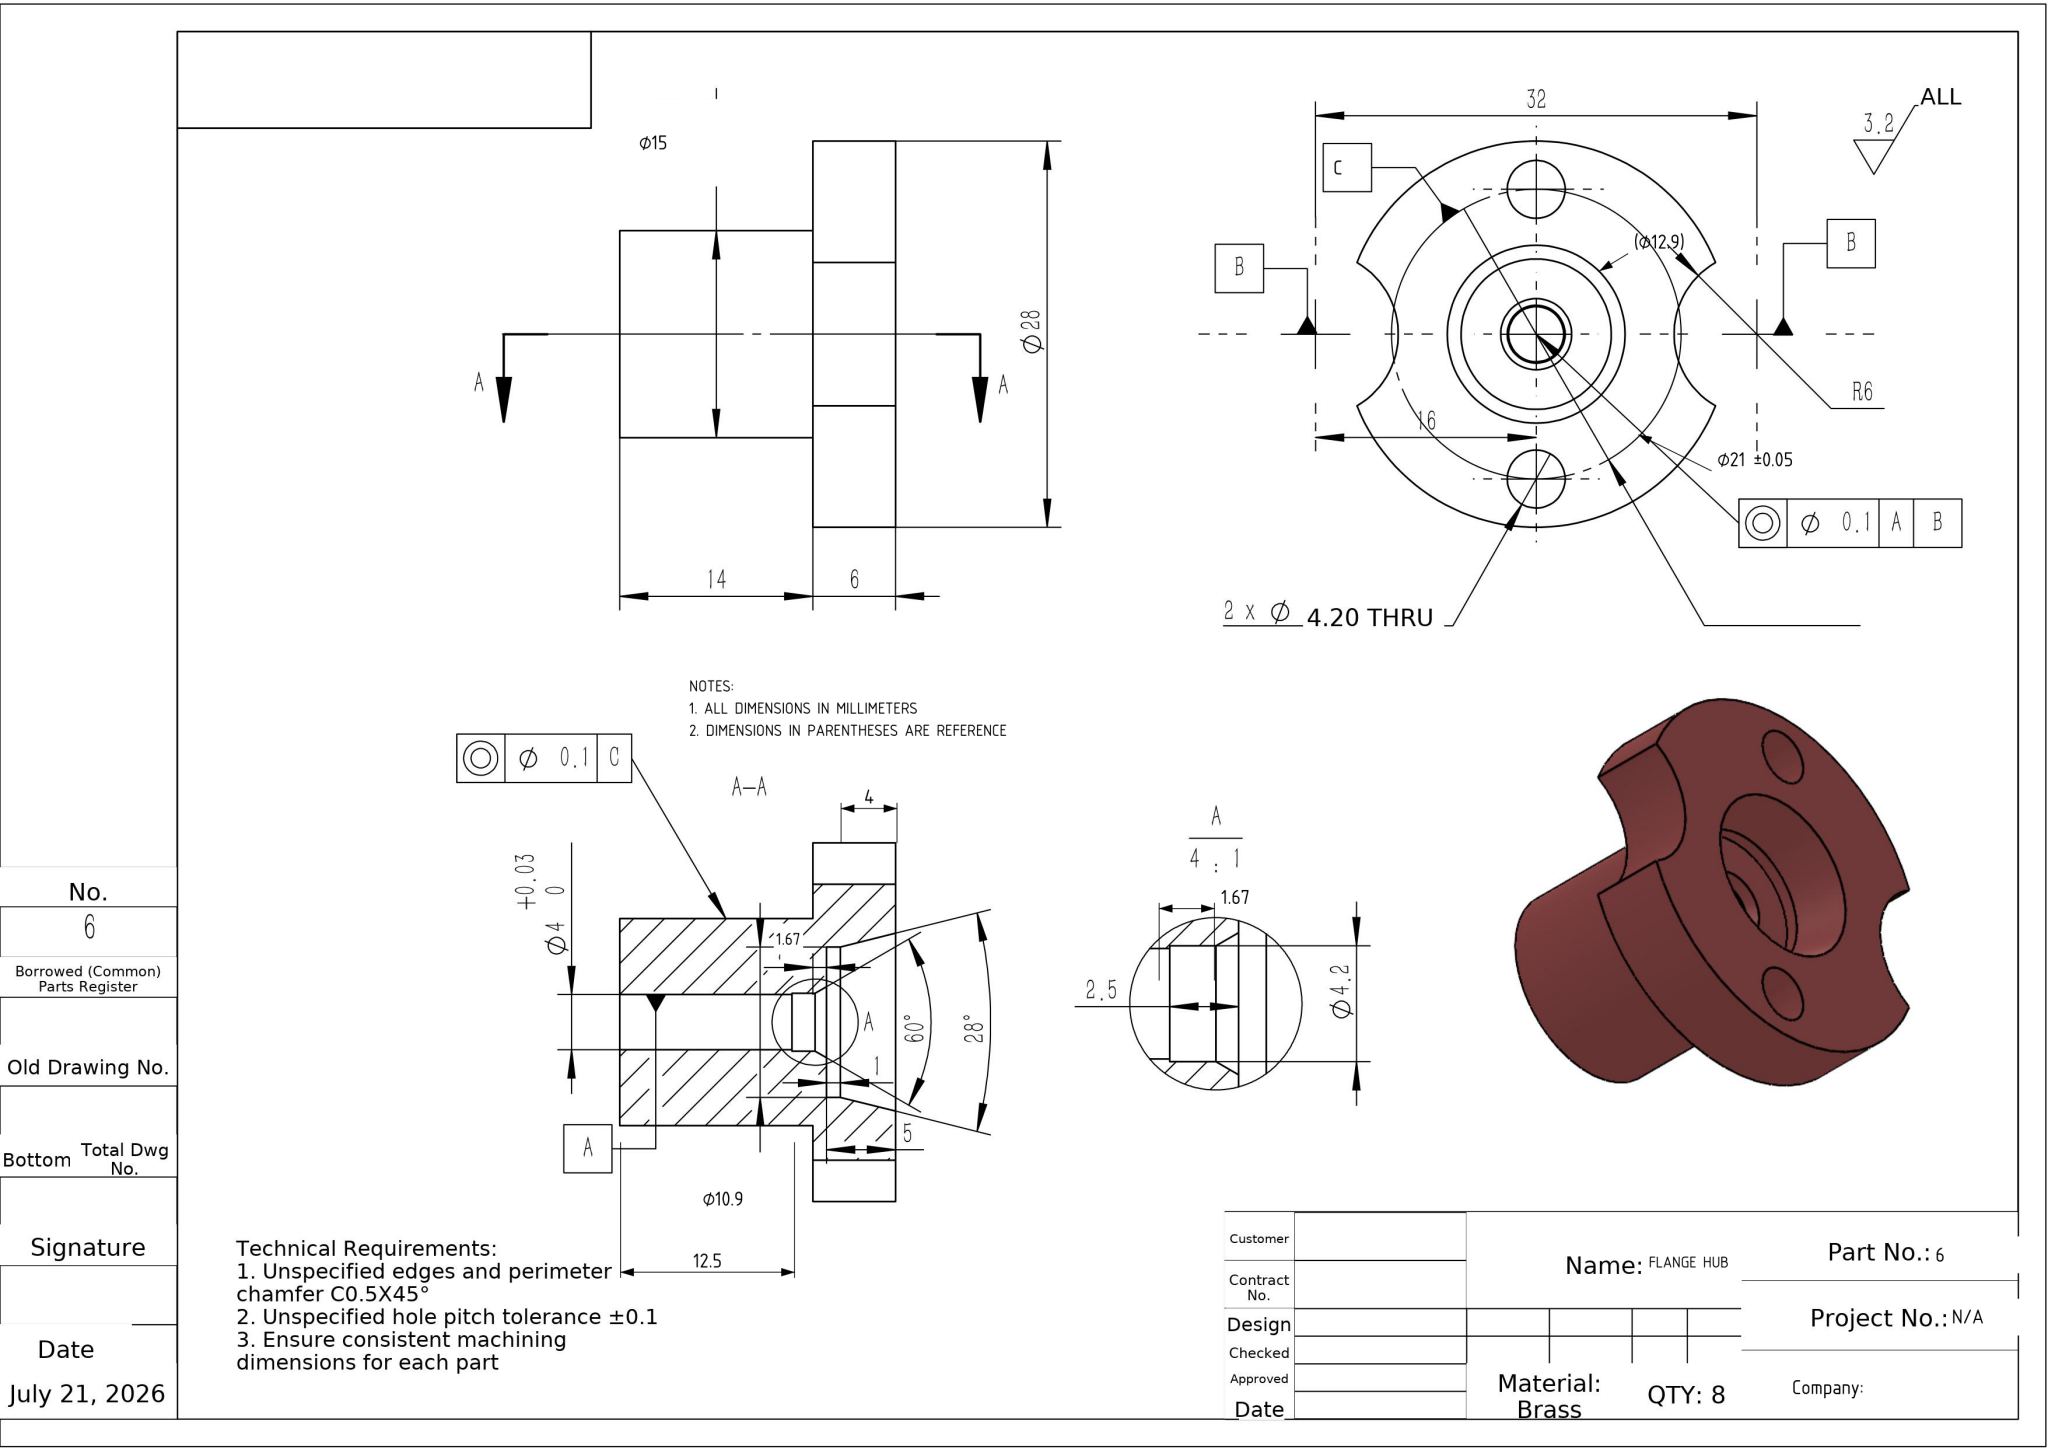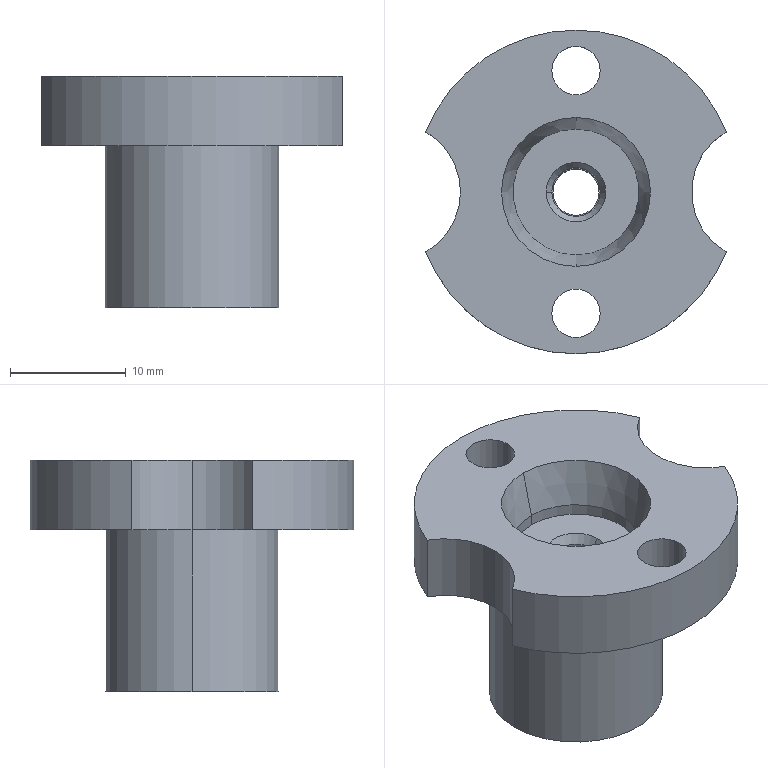Part | NX | mm | 1 solid | 26 faces | box 26 x 28 x 20 mm | volume 4920 mm3 | cylinder 17 | plane 5 | cone 4 | commonest cylinder face diameters 4.2 x6 12 x3 10.9 x2 15 x2 4 x2 28 x2
STEP:
#1=CARTESIAN_POINT('',(-2.1,0.,14.5));
#2=VERTEX_POINT('',#1);
#3=CARTESIAN_POINT('',(2.1,0.,14.5));
#4=VERTEX_POINT('',#3);
#5=CARTESIAN_POINT('',(0.,0.,14.5));
#6=DIRECTION('',(0.,0.,1.));
#7=DIRECTION('',(1.,0.,0.));
#8=AXIS2_PLACEMENT_3D('',#5,#6,#7);
#9=CIRCLE('',#8,2.1);
#10=EDGE_CURVE('',#2,#4,#9,.T.);
#11=ORIENTED_EDGE('',*,*,#10,.F.);
#12=CARTESIAN_POINT('',(-2.1,0.,16.173));
#13=VERTEX_POINT('',#12);
#14=CARTESIAN_POINT('',(-2.1,0.,14.5));
#15=DIRECTION('',(0.,0.,1.));
#16=VECTOR('',#15,1000.);
#17=LINE('',#14,#16);
#18=EDGE_CURVE('',#2,#13,#17,.T.);
#19=ORIENTED_EDGE('',*,*,#18,.T.);
#20=CARTESIAN_POINT('',(2.1,0.,16.173));
#21=VERTEX_POINT('',#20);
#22=CARTESIAN_POINT('',(0.,0.,16.173));
#23=DIRECTION('',(0.,0.,-1.));
#24=DIRECTION('',(1.,0.,0.));
#25=AXIS2_PLACEMENT_3D('',#22,#23,#24);
#26=CIRCLE('',#25,2.1);
#27=EDGE_CURVE('',#21,#13,#26,.T.);
#28=ORIENTED_EDGE('',*,*,#27,.F.);
#29=CARTESIAN_POINT('',(2.1,0.,14.5));
#30=DIRECTION('',(0.,0.,1.));
#31=VECTOR('',#30,1000.);
#32=LINE('',#29,#31);
#33=EDGE_CURVE('',#4,#21,#32,.T.);
#34=ORIENTED_EDGE('',*,*,#33,.F.);
#35=EDGE_LOOP('',(#11,#19,#28,#34));
#36=FACE_OUTER_BOUND('',#35,.T.);
#37=CARTESIAN_POINT('',(0.,0.,14.5));
#38=DIRECTION('',(0.,0.,1.));
#39=DIRECTION('',(1.,0.,0.));
#40=AXIS2_PLACEMENT_3D('',#37,#38,#39);
#41=CYLINDRICAL_SURFACE('',#40,2.1);
#42=ADVANCED_FACE('',(#36),#41,.F.);
#43=CARTESIAN_POINT('',(-13.,5.196,16.));
#44=VERTEX_POINT('',#43);
#45=CARTESIAN_POINT('',(-10.,0.,16.));
#46=VERTEX_POINT('',#45);
#47=CARTESIAN_POINT('',(-16.,0.,16.));
#48=DIRECTION('',(0.,0.,-1.));
#49=DIRECTION('',(-1.,0.,0.));
#50=AXIS2_PLACEMENT_3D('',#47,#48,#49);
#51=CIRCLE('',#50,6.);
#52=EDGE_CURVE('',#44,#46,#51,.T.);
#53=ORIENTED_EDGE('',*,*,#52,.T.);
#54=CARTESIAN_POINT('',(-10.,0.,22.));
#55=VERTEX_POINT('',#54);
#56=CARTESIAN_POINT('',(-10.,0.,0.));
#57=DIRECTION('',(0.,0.,1.));
#58=VECTOR('',#57,1000.);
#59=LINE('',#56,#58);
#60=EDGE_CURVE('',#46,#55,#59,.T.);
#61=ORIENTED_EDGE('',*,*,#60,.T.);
#62=CARTESIAN_POINT('',(-13.,5.196,22.));
#63=VERTEX_POINT('',#62);
#64=CARTESIAN_POINT('',(-16.,0.,22.));
#65=DIRECTION('',(0.,0.,1.));
#66=DIRECTION('',(1.,0.,0.));
#67=AXIS2_PLACEMENT_3D('',#64,#65,#66);
#68=CIRCLE('',#67,6.);
#69=EDGE_CURVE('',#55,#63,#68,.T.);
#70=ORIENTED_EDGE('',*,*,#69,.T.);
#71=CARTESIAN_POINT('',(-13.,5.196,11.));
#72=DIRECTION('',(0.,0.,1.));
#73=VECTOR('',#72,1000.);
#74=LINE('',#71,#73);
#75=EDGE_CURVE('',#44,#63,#74,.T.);
#76=ORIENTED_EDGE('',*,*,#75,.F.);
#77=EDGE_LOOP('',(#53,#61,#70,#76));
#78=FACE_OUTER_BOUND('',#77,.T.);
#79=CARTESIAN_POINT('',(-16.,0.,0.));
#80=DIRECTION('',(0.,0.,1.));
#81=DIRECTION('',(1.,0.,0.));
#82=AXIS2_PLACEMENT_3D('',#79,#80,#81);
#83=CYLINDRICAL_SURFACE('',#82,6.);
#84=ADVANCED_FACE('',(#78),#83,.F.);
#85=CARTESIAN_POINT('',(2.1,10.5,16.));
#86=VERTEX_POINT('',#85);
#87=CARTESIAN_POINT('',(-2.1,10.5,16.));
#88=VERTEX_POINT('',#87);
#89=CARTESIAN_POINT('',(0.,10.5,16.));
#90=DIRECTION('',(0.,0.,-1.));
#91=DIRECTION('',(-1.,0.,0.));
#92=AXIS2_PLACEMENT_3D('',#89,#90,#91);
#93=CIRCLE('',#92,2.1);
#94=EDGE_CURVE('',#86,#88,#93,.T.);
#95=ORIENTED_EDGE('',*,*,#94,.T.);
#96=CARTESIAN_POINT('',(-2.1,10.5,22.));
#97=VERTEX_POINT('',#96);
#98=CARTESIAN_POINT('',(-2.1,10.5,22.));
#99=DIRECTION('',(0.,0.,1.));
#100=VECTOR('',#99,1000.);
#101=LINE('',#98,#100);
#102=EDGE_CURVE('',#88,#97,#101,.T.);
#103=ORIENTED_EDGE('',*,*,#102,.T.);
#104=CARTESIAN_POINT('',(2.1,10.5,22.));
#105=VERTEX_POINT('',#104);
#106=CARTESIAN_POINT('',(0.,10.5,22.));
#107=DIRECTION('',(0.,0.,1.));
#108=DIRECTION('',(1.,0.,0.));
#109=AXIS2_PLACEMENT_3D('',#106,#107,#108);
#110=CIRCLE('',#109,2.1);
#111=EDGE_CURVE('',#97,#105,#110,.T.);
#112=ORIENTED_EDGE('',*,*,#111,.T.);
#113=CARTESIAN_POINT('',(2.1,10.5,22.));
#114=DIRECTION('',(0.,0.,1.));
#115=VECTOR('',#114,1000.);
#116=LINE('',#113,#115);
#117=EDGE_CURVE('',#86,#105,#116,.T.);
#118=ORIENTED_EDGE('',*,*,#117,.F.);
#119=EDGE_LOOP('',(#95,#103,#112,#118));
#120=FACE_OUTER_BOUND('',#119,.T.);
#121=CARTESIAN_POINT('',(0.,10.5,22.));
#122=DIRECTION('',(0.,0.,1.));
#123=DIRECTION('',(1.,0.,0.));
#124=AXIS2_PLACEMENT_3D('',#121,#122,#123);
#125=CYLINDRICAL_SURFACE('',#124,2.1);
#126=ADVANCED_FACE('',(#120),#125,.F.);
#127=CARTESIAN_POINT('',(2.1,-10.5,16.));
#128=VERTEX_POINT('',#127);
#129=CARTESIAN_POINT('',(-2.1,-10.5,16.));
#130=VERTEX_POINT('',#129);
#131=CARTESIAN_POINT('',(0.,-10.5,16.));
#132=DIRECTION('',(0.,0.,-1.));
#133=DIRECTION('',(-1.,0.,0.));
#134=AXIS2_PLACEMENT_3D('',#131,#132,#133);
#135=CIRCLE('',#134,2.1);
#136=EDGE_CURVE('',#128,#130,#135,.T.);
#137=ORIENTED_EDGE('',*,*,#136,.T.);
#138=CARTESIAN_POINT('',(-2.1,-10.5,22.));
#139=VERTEX_POINT('',#138);
#140=CARTESIAN_POINT('',(-2.1,-10.5,22.));
#141=DIRECTION('',(0.,0.,1.));
#142=VECTOR('',#141,1000.);
#143=LINE('',#140,#142);
#144=EDGE_CURVE('',#130,#139,#143,.T.);
#145=ORIENTED_EDGE('',*,*,#144,.T.);
#146=CARTESIAN_POINT('',(2.1,-10.5,22.));
#147=VERTEX_POINT('',#146);
#148=CARTESIAN_POINT('',(0.,-10.5,22.));
#149=DIRECTION('',(0.,0.,1.));
#150=DIRECTION('',(1.,0.,0.));
#151=AXIS2_PLACEMENT_3D('',#148,#149,#150);
#152=CIRCLE('',#151,2.1);
#153=EDGE_CURVE('',#139,#147,#152,.T.);
#154=ORIENTED_EDGE('',*,*,#153,.T.);
#155=CARTESIAN_POINT('',(2.1,-10.5,22.));
#156=DIRECTION('',(0.,0.,1.));
#157=VECTOR('',#156,1000.);
#158=LINE('',#155,#157);
#159=EDGE_CURVE('',#128,#147,#158,.T.);
#160=ORIENTED_EDGE('',*,*,#159,.F.);
#161=EDGE_LOOP('',(#137,#145,#154,#160));
#162=FACE_OUTER_BOUND('',#161,.T.);
#163=CARTESIAN_POINT('',(0.,-10.5,22.));
#164=DIRECTION('',(0.,0.,1.));
#165=DIRECTION('',(1.,0.,0.));
#166=AXIS2_PLACEMENT_3D('',#163,#164,#165);
#167=CYLINDRICAL_SURFACE('',#166,2.1);
#168=ADVANCED_FACE('',(#162),#167,.F.);
#169=CARTESIAN_POINT('',(0.,-5.45,18.));
#170=VERTEX_POINT('',#169);
#171=CARTESIAN_POINT('',(0.,5.45,18.));
#172=VERTEX_POINT('',#171);
#173=CARTESIAN_POINT('',(0.,-0.,18.));
#174=DIRECTION('',(0.,0.,-1.));
#175=DIRECTION('',(0.,1.,0.));
#176=AXIS2_PLACEMENT_3D('',#173,#174,#175);
#177=CIRCLE('',#176,5.45);
#178=EDGE_CURVE('',#170,#172,#177,.T.);
#179=ORIENTED_EDGE('',*,*,#178,.F.);
#180=CARTESIAN_POINT('',(0.,-5.45,17.));
#181=VERTEX_POINT('',#180);
#182=CARTESIAN_POINT('',(0.,-5.45,-0.));
#183=DIRECTION('',(0.,0.,-1.));
#184=VECTOR('',#183,1000.);
#185=LINE('',#182,#184);
#186=EDGE_CURVE('',#170,#181,#185,.T.);
#187=ORIENTED_EDGE('',*,*,#186,.T.);
#188=CARTESIAN_POINT('',(0.,5.45,17.));
#189=VERTEX_POINT('',#188);
#190=CARTESIAN_POINT('',(0.,-0.,17.));
#191=DIRECTION('',(0.,0.,-1.));
#192=DIRECTION('',(0.,1.,0.));
#193=AXIS2_PLACEMENT_3D('',#190,#191,#192);
#194=CIRCLE('',#193,5.45);
#195=EDGE_CURVE('',#181,#189,#194,.T.);
#196=ORIENTED_EDGE('',*,*,#195,.T.);
#197=CARTESIAN_POINT('',(0.,5.45,0.));
#198=DIRECTION('',(0.,0.,-1.));
#199=VECTOR('',#198,1000.);
#200=LINE('',#197,#199);
#201=EDGE_CURVE('',#172,#189,#200,.T.);
#202=ORIENTED_EDGE('',*,*,#201,.F.);
#203=EDGE_LOOP('',(#179,#187,#196,#202));
#204=FACE_OUTER_BOUND('',#203,.T.);
#205=CARTESIAN_POINT('',(0.,0.,0.));
#206=DIRECTION('',(0.,0.,-1.));
#207=DIRECTION('',(0.,1.,0.));
#208=AXIS2_PLACEMENT_3D('',#205,#206,#207);
#209=CYLINDRICAL_SURFACE('',#208,5.45);
#210=ADVANCED_FACE('',(#204),#209,.F.);
#211=ORIENTED_EDGE('',*,*,#178,.T.);
#212=CARTESIAN_POINT('',(0.,6.447,22.));
#213=VERTEX_POINT('',#212);
#214=CARTESIAN_POINT('',(0.,5.45,18.));
#215=DIRECTION('',(0.,0.2419,0.9703));
#216=VECTOR('',#215,1000.);
#217=LINE('',#214,#216);
#218=EDGE_CURVE('',#172,#213,#217,.T.);
#219=ORIENTED_EDGE('',*,*,#218,.T.);
#220=CARTESIAN_POINT('',(0.,-6.447,22.));
#221=VERTEX_POINT('',#220);
#222=CARTESIAN_POINT('',(0.,-0.,22.));
#223=DIRECTION('',(0.,0.,1.));
#224=DIRECTION('',(1.,0.,0.));
#225=AXIS2_PLACEMENT_3D('',#222,#223,#224);
#226=CIRCLE('',#225,6.447);
#227=EDGE_CURVE('',#213,#221,#226,.T.);
#228=ORIENTED_EDGE('',*,*,#227,.T.);
#229=CARTESIAN_POINT('',(0.,-5.45,18.));
#230=DIRECTION('',(0.,-0.2419,0.9703));
#231=VECTOR('',#230,1000.);
#232=LINE('',#229,#231);
#233=EDGE_CURVE('',#170,#221,#232,.T.);
#234=ORIENTED_EDGE('',*,*,#233,.F.);
#235=EDGE_LOOP('',(#211,#219,#228,#234));
#236=FACE_OUTER_BOUND('',#235,.T.);
#237=CARTESIAN_POINT('',(0.,-0.,18.));
#238=DIRECTION('',(0.,-0.,1.));
#239=DIRECTION('',(0.,-1.,0.));
#240=AXIS2_PLACEMENT_3D('',#237,#238,#239);
#241=CONICAL_SURFACE('',#240,5.45,0.2443);
#242=ADVANCED_FACE('',(#236),#241,.F.);
#243=ORIENTED_EDGE('',*,*,#27,.T.);
#244=CARTESIAN_POINT('',(-2.577,0.,17.));
#245=VERTEX_POINT('',#244);
#246=CARTESIAN_POINT('',(-2.,0.,16.));
#247=DIRECTION('',(-0.5,0.,0.866));
#248=VECTOR('',#247,1000.);
#249=LINE('',#246,#248);
#250=EDGE_CURVE('',#13,#245,#249,.T.);
#251=ORIENTED_EDGE('',*,*,#250,.T.);
#252=CARTESIAN_POINT('',(2.577,0.,17.));
#253=VERTEX_POINT('',#252);
#254=CARTESIAN_POINT('',(0.,0.,17.));
#255=DIRECTION('',(0.,-0.,1.));
#256=DIRECTION('',(0.,1.,0.));
#257=AXIS2_PLACEMENT_3D('',#254,#255,#256);
#258=CIRCLE('',#257,2.577);
#259=EDGE_CURVE('',#245,#253,#258,.T.);
#260=ORIENTED_EDGE('',*,*,#259,.T.);
#261=CARTESIAN_POINT('',(2.,0.,16.));
#262=DIRECTION('',(0.5,0.,0.866));
#263=VECTOR('',#262,1000.);
#264=LINE('',#261,#263);
#265=EDGE_CURVE('',#21,#253,#264,.T.);
#266=ORIENTED_EDGE('',*,*,#265,.F.);
#267=EDGE_LOOP('',(#243,#251,#260,#266));
#268=FACE_OUTER_BOUND('',#267,.T.);
#269=CARTESIAN_POINT('',(0.,0.,16.));
#270=DIRECTION('',(0.,0.,1.));
#271=DIRECTION('',(1.,0.,0.));
#272=AXIS2_PLACEMENT_3D('',#269,#270,#271);
#273=CONICAL_SURFACE('',#272,2.,0.5236);
#274=ADVANCED_FACE('',(#268),#273,.F.);
#275=CARTESIAN_POINT('',(-7.5,0.,16.));
#276=VERTEX_POINT('',#275);
#277=CARTESIAN_POINT('',(7.5,0.,16.));
#278=VERTEX_POINT('',#277);
#279=CARTESIAN_POINT('',(0.,0.,16.));
#280=DIRECTION('',(0.,0.,-1.));
#281=DIRECTION('',(-1.,0.,0.));
#282=AXIS2_PLACEMENT_3D('',#279,#280,#281);
#283=CIRCLE('',#282,7.5);
#284=EDGE_CURVE('',#276,#278,#283,.T.);
#285=ORIENTED_EDGE('',*,*,#284,.T.);
#286=CARTESIAN_POINT('',(7.5,0.,2.));
#287=VERTEX_POINT('',#286);
#288=CARTESIAN_POINT('',(7.5,0.,16.));
#289=DIRECTION('',(0.,0.,-1.));
#290=VECTOR('',#289,1000.);
#291=LINE('',#288,#290);
#292=EDGE_CURVE('',#278,#287,#291,.T.);
#293=ORIENTED_EDGE('',*,*,#292,.T.);
#294=CARTESIAN_POINT('',(-7.5,0.,2.));
#295=VERTEX_POINT('',#294);
#296=CARTESIAN_POINT('',(0.,0.,2.));
#297=DIRECTION('',(0.,0.,-1.));
#298=DIRECTION('',(-1.,0.,0.));
#299=AXIS2_PLACEMENT_3D('',#296,#297,#298);
#300=CIRCLE('',#299,7.5);
#301=EDGE_CURVE('',#295,#287,#300,.T.);
#302=ORIENTED_EDGE('',*,*,#301,.F.);
#303=CARTESIAN_POINT('',(-7.5,0.,16.));
#304=DIRECTION('',(0.,0.,-1.));
#305=VECTOR('',#304,1000.);
#306=LINE('',#303,#305);
#307=EDGE_CURVE('',#276,#295,#306,.T.);
#308=ORIENTED_EDGE('',*,*,#307,.F.);
#309=EDGE_LOOP('',(#285,#293,#302,#308));
#310=FACE_OUTER_BOUND('',#309,.T.);
#311=CARTESIAN_POINT('',(0.,0.,16.));
#312=DIRECTION('',(0.,0.,-1.));
#313=DIRECTION('',(-1.,0.,0.));
#314=AXIS2_PLACEMENT_3D('',#311,#312,#313);
#315=CYLINDRICAL_SURFACE('',#314,7.5);
#316=ADVANCED_FACE('',(#310),#315,.T.);
#317=CARTESIAN_POINT('',(2.,0.,14.5));
#318=VERTEX_POINT('',#317);
#319=CARTESIAN_POINT('',(-2.,0.,14.5));
#320=VERTEX_POINT('',#319);
#321=CARTESIAN_POINT('',(0.,0.,14.5));
#322=DIRECTION('',(0.,0.,-1.));
#323=DIRECTION('',(1.,0.,0.));
#324=AXIS2_PLACEMENT_3D('',#321,#322,#323);
#325=CIRCLE('',#324,2.);
#326=EDGE_CURVE('',#318,#320,#325,.T.);
#327=ORIENTED_EDGE('',*,*,#326,.F.);
#328=CARTESIAN_POINT('',(2.,0.,2.));
#329=VERTEX_POINT('',#328);
#330=CARTESIAN_POINT('',(2.,0.,0.));
#331=DIRECTION('',(0.,0.,-1.));
#332=VECTOR('',#331,1000.);
#333=LINE('',#330,#332);
#334=EDGE_CURVE('',#318,#329,#333,.T.);
#335=ORIENTED_EDGE('',*,*,#334,.T.);
#336=CARTESIAN_POINT('',(-2.,0.,2.));
#337=VERTEX_POINT('',#336);
#338=CARTESIAN_POINT('',(0.,0.,2.));
#339=DIRECTION('',(0.,0.,-1.));
#340=DIRECTION('',(-1.,0.,0.));
#341=AXIS2_PLACEMENT_3D('',#338,#339,#340);
#342=CIRCLE('',#341,2.);
#343=EDGE_CURVE('',#329,#337,#342,.T.);
#344=ORIENTED_EDGE('',*,*,#343,.T.);
#345=CARTESIAN_POINT('',(-2.,0.,0.));
#346=DIRECTION('',(0.,0.,-1.));
#347=VECTOR('',#346,1000.);
#348=LINE('',#345,#347);
#349=EDGE_CURVE('',#320,#337,#348,.T.);
#350=ORIENTED_EDGE('',*,*,#349,.F.);
#351=EDGE_LOOP('',(#327,#335,#344,#350));
#352=FACE_OUTER_BOUND('',#351,.T.);
#353=CARTESIAN_POINT('',(0.,0.,0.));
#354=DIRECTION('',(0.,0.,-1.));
#355=DIRECTION('',(-1.,0.,0.));
#356=AXIS2_PLACEMENT_3D('',#353,#354,#355);
#357=CYLINDRICAL_SURFACE('',#356,2.);
#358=ADVANCED_FACE('',(#352),#357,.F.);
#359=ORIENTED_EDGE('',*,*,#334,.F.);
#360=CARTESIAN_POINT('',(0.,0.,14.5));
#361=DIRECTION('',(0.,0.,-1.));
#362=DIRECTION('',(1.,0.,0.));
#363=AXIS2_PLACEMENT_3D('',#360,#361,#362);
#364=CIRCLE('',#363,2.);
#365=EDGE_CURVE('',#320,#318,#364,.T.);
#366=ORIENTED_EDGE('',*,*,#365,.F.);
#367=ORIENTED_EDGE('',*,*,#349,.T.);
#368=CARTESIAN_POINT('',(0.,0.,2.));
#369=DIRECTION('',(0.,0.,-1.));
#370=DIRECTION('',(-1.,0.,0.));
#371=AXIS2_PLACEMENT_3D('',#368,#369,#370);
#372=CIRCLE('',#371,2.);
#373=EDGE_CURVE('',#337,#329,#372,.T.);
#374=ORIENTED_EDGE('',*,*,#373,.T.);
#375=EDGE_LOOP('',(#359,#366,#367,#374));
#376=FACE_OUTER_BOUND('',#375,.T.);
#377=CARTESIAN_POINT('',(0.,0.,0.));
#378=DIRECTION('',(0.,0.,-1.));
#379=DIRECTION('',(-1.,0.,0.));
#380=AXIS2_PLACEMENT_3D('',#377,#378,#379);
#381=CYLINDRICAL_SURFACE('',#380,2.);
#382=ADVANCED_FACE('',(#376),#381,.F.);
#383=ORIENTED_EDGE('',*,*,#292,.F.);
#384=CARTESIAN_POINT('',(0.,0.,16.));
#385=DIRECTION('',(0.,0.,-1.));
#386=DIRECTION('',(-1.,0.,0.));
#387=AXIS2_PLACEMENT_3D('',#384,#385,#386);
#388=CIRCLE('',#387,7.5);
#389=EDGE_CURVE('',#278,#276,#388,.T.);
#390=ORIENTED_EDGE('',*,*,#389,.T.);
#391=ORIENTED_EDGE('',*,*,#307,.T.);
#392=CARTESIAN_POINT('',(0.,0.,2.));
#393=DIRECTION('',(0.,0.,-1.));
#394=DIRECTION('',(-1.,0.,0.));
#395=AXIS2_PLACEMENT_3D('',#392,#393,#394);
#396=CIRCLE('',#395,7.5);
#397=EDGE_CURVE('',#287,#295,#396,.T.);
#398=ORIENTED_EDGE('',*,*,#397,.F.);
#399=EDGE_LOOP('',(#383,#390,#391,#398));
#400=FACE_OUTER_BOUND('',#399,.T.);
#401=CARTESIAN_POINT('',(0.,0.,16.));
#402=DIRECTION('',(0.,0.,-1.));
#403=DIRECTION('',(-1.,0.,0.));
#404=AXIS2_PLACEMENT_3D('',#401,#402,#403);
#405=CYLINDRICAL_SURFACE('',#404,7.5);
#406=ADVANCED_FACE('',(#400),#405,.T.);
#407=CARTESIAN_POINT('',(13.,-5.196,16.));
#408=VERTEX_POINT('',#407);
#409=CARTESIAN_POINT('',(-13.,-5.196,16.));
#410=VERTEX_POINT('',#409);
#411=CARTESIAN_POINT('',(0.,0.,16.));
#412=DIRECTION('',(0.,0.,-1.));
#413=DIRECTION('',(-1.,0.,0.));
#414=AXIS2_PLACEMENT_3D('',#411,#412,#413);
#415=CIRCLE('',#414,14.);
#416=EDGE_CURVE('',#408,#410,#415,.T.);
#417=ORIENTED_EDGE('',*,*,#416,.F.);
#418=CARTESIAN_POINT('',(13.,-5.196,22.));
#419=VERTEX_POINT('',#418);
#420=CARTESIAN_POINT('',(13.,-5.196,11.));
#421=DIRECTION('',(0.,0.,1.));
#422=VECTOR('',#421,1000.);
#423=LINE('',#420,#422);
#424=EDGE_CURVE('',#408,#419,#423,.T.);
#425=ORIENTED_EDGE('',*,*,#424,.T.);
#426=CARTESIAN_POINT('',(-13.,-5.196,22.));
#427=VERTEX_POINT('',#426);
#428=CARTESIAN_POINT('',(0.,0.,22.));
#429=DIRECTION('',(0.,0.,1.));
#430=DIRECTION('',(1.,0.,0.));
#431=AXIS2_PLACEMENT_3D('',#428,#429,#430);
#432=CIRCLE('',#431,14.);
#433=EDGE_CURVE('',#427,#419,#432,.T.);
#434=ORIENTED_EDGE('',*,*,#433,.F.);
#435=CARTESIAN_POINT('',(-13.,-5.196,11.));
#436=DIRECTION('',(0.,0.,-1.));
#437=VECTOR('',#436,1000.);
#438=LINE('',#435,#437);
#439=EDGE_CURVE('',#427,#410,#438,.T.);
#440=ORIENTED_EDGE('',*,*,#439,.T.);
#441=EDGE_LOOP('',(#417,#425,#434,#440));
#442=FACE_OUTER_BOUND('',#441,.T.);
#443=CARTESIAN_POINT('',(0.,0.,22.));
#444=DIRECTION('',(0.,0.,-1.));
#445=DIRECTION('',(-1.,0.,0.));
#446=AXIS2_PLACEMENT_3D('',#443,#444,#445);
#447=CYLINDRICAL_SURFACE('',#446,14.);
#448=ADVANCED_FACE('',(#442),#447,.T.);
#449=CARTESIAN_POINT('',(13.,5.196,22.));
#450=VERTEX_POINT('',#449);
#451=CARTESIAN_POINT('',(0.,0.,22.));
#452=DIRECTION('',(0.,0.,1.));
#453=DIRECTION('',(1.,0.,0.));
#454=AXIS2_PLACEMENT_3D('',#451,#452,#453);
#455=CIRCLE('',#454,14.);
#456=EDGE_CURVE('',#450,#63,#455,.T.);
#457=ORIENTED_EDGE('',*,*,#456,.F.);
#458=CARTESIAN_POINT('',(13.,5.196,16.));
#459=VERTEX_POINT('',#458);
#460=CARTESIAN_POINT('',(13.,5.196,11.));
#461=DIRECTION('',(0.,0.,-1.));
#462=VECTOR('',#461,1000.);
#463=LINE('',#460,#462);
#464=EDGE_CURVE('',#450,#459,#463,.T.);
#465=ORIENTED_EDGE('',*,*,#464,.T.);
#466=CARTESIAN_POINT('',(0.,0.,16.));
#467=DIRECTION('',(0.,0.,-1.));
#468=DIRECTION('',(-1.,0.,0.));
#469=AXIS2_PLACEMENT_3D('',#466,#467,#468);
#470=CIRCLE('',#469,14.);
#471=EDGE_CURVE('',#44,#459,#470,.T.);
#472=ORIENTED_EDGE('',*,*,#471,.F.);
#473=ORIENTED_EDGE('',*,*,#75,.T.);
#474=EDGE_LOOP('',(#457,#465,#472,#473));
#475=FACE_OUTER_BOUND('',#474,.T.);
#476=CARTESIAN_POINT('',(0.,0.,22.));
#477=DIRECTION('',(0.,0.,-1.));
#478=DIRECTION('',(-1.,0.,0.));
#479=AXIS2_PLACEMENT_3D('',#476,#477,#478);
#480=CYLINDRICAL_SURFACE('',#479,14.);
#481=ADVANCED_FACE('',(#475),#480,.T.);
#482=CARTESIAN_POINT('',(16.,0.,22.));
#483=DIRECTION('',(0.,0.,1.));
#484=DIRECTION('',(1.,0.,0.));
#485=AXIS2_PLACEMENT_3D('',#482,#483,#484);
#486=CIRCLE('',#485,6.);
#487=EDGE_CURVE('',#450,#419,#486,.T.);
#488=ORIENTED_EDGE('',*,*,#487,.F.);
#489=ORIENTED_EDGE('',*,*,#456,.T.);
#490=ORIENTED_EDGE('',*,*,#69,.F.);
#491=CARTESIAN_POINT('',(-16.,0.,22.));
#492=DIRECTION('',(0.,0.,1.));
#493=DIRECTION('',(1.,0.,0.));
#494=AXIS2_PLACEMENT_3D('',#491,#492,#493);
#495=CIRCLE('',#494,6.);
#496=EDGE_CURVE('',#427,#55,#495,.T.);
#497=ORIENTED_EDGE('',*,*,#496,.F.);
#498=ORIENTED_EDGE('',*,*,#433,.T.);
#499=EDGE_LOOP('',(#488,#489,#490,#497,#498));
#500=FACE_OUTER_BOUND('',#499,.T.);
#501=CARTESIAN_POINT('',(0.,10.5,22.));
#502=DIRECTION('',(0.,0.,1.));
#503=DIRECTION('',(1.,0.,0.));
#504=AXIS2_PLACEMENT_3D('',#501,#502,#503);
#505=CIRCLE('',#504,2.1);
#506=EDGE_CURVE('',#105,#97,#505,.T.);
#507=ORIENTED_EDGE('',*,*,#506,.F.);
#508=ORIENTED_EDGE('',*,*,#111,.F.);
#509=EDGE_LOOP('',(#507,#508));
#510=FACE_BOUND('',#509,.T.);
#511=CARTESIAN_POINT('',(0.,-10.5,22.));
#512=DIRECTION('',(0.,0.,1.));
#513=DIRECTION('',(1.,0.,0.));
#514=AXIS2_PLACEMENT_3D('',#511,#512,#513);
#515=CIRCLE('',#514,2.1);
#516=EDGE_CURVE('',#147,#139,#515,.T.);
#517=ORIENTED_EDGE('',*,*,#516,.F.);
#518=ORIENTED_EDGE('',*,*,#153,.F.);
#519=EDGE_LOOP('',(#517,#518));
#520=FACE_BOUND('',#519,.T.);
#521=CARTESIAN_POINT('',(0.,-0.,22.));
#522=DIRECTION('',(0.,0.,1.));
#523=DIRECTION('',(1.,0.,0.));
#524=AXIS2_PLACEMENT_3D('',#521,#522,#523);
#525=CIRCLE('',#524,6.447);
#526=EDGE_CURVE('',#221,#213,#525,.T.);
#527=ORIENTED_EDGE('',*,*,#526,.F.);
#528=ORIENTED_EDGE('',*,*,#227,.F.);
#529=EDGE_LOOP('',(#527,#528));
#530=FACE_BOUND('',#529,.T.);
#531=CARTESIAN_POINT('',(0.,0.,22.));
#532=DIRECTION('',(0.,0.,1.));
#533=DIRECTION('',(1.,0.,0.));
#534=AXIS2_PLACEMENT_3D('',#531,#532,#533);
#535=PLANE('',#534);
#536=ADVANCED_FACE('',(#500,#510,#520,#530),#535,.T.);
#537=CARTESIAN_POINT('',(16.,0.,16.));
#538=DIRECTION('',(0.,0.,-1.));
#539=DIRECTION('',(-1.,0.,0.));
#540=AXIS2_PLACEMENT_3D('',#537,#538,#539);
#541=CIRCLE('',#540,6.);
#542=EDGE_CURVE('',#408,#459,#541,.T.);
#543=ORIENTED_EDGE('',*,*,#542,.F.);
#544=ORIENTED_EDGE('',*,*,#416,.T.);
#545=CARTESIAN_POINT('',(-16.,0.,16.));
#546=DIRECTION('',(0.,0.,-1.));
#547=DIRECTION('',(-1.,0.,0.));
#548=AXIS2_PLACEMENT_3D('',#545,#546,#547);
#549=CIRCLE('',#548,6.);
#550=EDGE_CURVE('',#46,#410,#549,.T.);
#551=ORIENTED_EDGE('',*,*,#550,.F.);
#552=ORIENTED_EDGE('',*,*,#52,.F.);
#553=ORIENTED_EDGE('',*,*,#471,.T.);
#554=EDGE_LOOP('',(#543,#544,#551,#552,#553));
#555=FACE_OUTER_BOUND('',#554,.T.);
#556=ORIENTED_EDGE('',*,*,#94,.F.);
#557=CARTESIAN_POINT('',(0.,10.5,16.));
#558=DIRECTION('',(0.,0.,-1.));
#559=DIRECTION('',(-1.,0.,0.));
#560=AXIS2_PLACEMENT_3D('',#557,#558,#559);
#561=CIRCLE('',#560,2.1);
#562=EDGE_CURVE('',#88,#86,#561,.T.);
#563=ORIENTED_EDGE('',*,*,#562,.F.);
#564=EDGE_LOOP('',(#556,#563));
#565=FACE_BOUND('',#564,.T.);
#566=ORIENTED_EDGE('',*,*,#136,.F.);
#567=CARTESIAN_POINT('',(0.,-10.5,16.));
#568=DIRECTION('',(0.,0.,-1.));
#569=DIRECTION('',(-1.,0.,0.));
#570=AXIS2_PLACEMENT_3D('',#567,#568,#569);
#571=CIRCLE('',#570,2.1);
#572=EDGE_CURVE('',#130,#128,#571,.T.);
#573=ORIENTED_EDGE('',*,*,#572,.F.);
#574=EDGE_LOOP('',(#566,#573));
#575=FACE_BOUND('',#574,.T.);
#576=ORIENTED_EDGE('',*,*,#284,.F.);
#577=ORIENTED_EDGE('',*,*,#389,.F.);
#578=EDGE_LOOP('',(#576,#577));
#579=FACE_BOUND('',#578,.T.);
#580=CARTESIAN_POINT('',(0.,0.,16.));
#581=DIRECTION('',(0.,0.,-1.));
#582=DIRECTION('',(-1.,0.,0.));
#583=AXIS2_PLACEMENT_3D('',#580,#581,#582);
#584=PLANE('',#583);
#585=ADVANCED_FACE('',(#555,#565,#575,#579),#584,.T.);
#586=ORIENTED_EDGE('',*,*,#250,.F.);
#587=CARTESIAN_POINT('',(0.,0.,16.173));
#588=DIRECTION('',(0.,0.,-1.));
#589=DIRECTION('',(1.,0.,0.));
#590=AXIS2_PLACEMENT_3D('',#587,#588,#589);
#591=CIRCLE('',#590,2.1);
#592=EDGE_CURVE('',#13,#21,#591,.T.);
#593=ORIENTED_EDGE('',*,*,#592,.T.);
#594=ORIENTED_EDGE('',*,*,#265,.T.);
#595=CARTESIAN_POINT('',(0.,0.,17.));
#596=DIRECTION('',(0.,-0.,1.));
#597=DIRECTION('',(0.,1.,0.));
#598=AXIS2_PLACEMENT_3D('',#595,#596,#597);
#599=CIRCLE('',#598,2.577);
#600=EDGE_CURVE('',#253,#245,#599,.T.);
#601=ORIENTED_EDGE('',*,*,#600,.T.);
#602=EDGE_LOOP('',(#586,#593,#594,#601));
#603=FACE_OUTER_BOUND('',#602,.T.);
#604=CARTESIAN_POINT('',(0.,0.,16.));
#605=DIRECTION('',(0.,0.,1.));
#606=DIRECTION('',(1.,0.,0.));
#607=AXIS2_PLACEMENT_3D('',#604,#605,#606);
#608=CONICAL_SURFACE('',#607,2.,0.5236);
#609=ADVANCED_FACE('',(#603),#608,.F.);
#610=CARTESIAN_POINT('',(0.,-0.,17.));
#611=DIRECTION('',(0.,0.,-1.));
#612=DIRECTION('',(0.,1.,0.));
#613=AXIS2_PLACEMENT_3D('',#610,#611,#612);
#614=CIRCLE('',#613,5.45);
#615=EDGE_CURVE('',#189,#181,#614,.T.);
#616=ORIENTED_EDGE('',*,*,#615,.F.);
#617=ORIENTED_EDGE('',*,*,#195,.F.);
#618=EDGE_LOOP('',(#616,#617));
#619=FACE_OUTER_BOUND('',#618,.T.);
#620=ORIENTED_EDGE('',*,*,#600,.F.);
#621=ORIENTED_EDGE('',*,*,#259,.F.);
#622=EDGE_LOOP('',(#620,#621));
#623=FACE_BOUND('',#622,.T.);
#624=CARTESIAN_POINT('',(0.,5.45,17.));
#625=DIRECTION('',(0.,0.,-1.));
#626=DIRECTION('',(0.,1.,0.));
#627=AXIS2_PLACEMENT_3D('',#624,#625,#626);
#628=PLANE('',#627);
#629=ADVANCED_FACE('',(#619,#623),#628,.F.);
#630=ORIENTED_EDGE('',*,*,#218,.F.);
#631=CARTESIAN_POINT('',(0.,-0.,18.));
#632=DIRECTION('',(0.,0.,-1.));
#633=DIRECTION('',(0.,1.,0.));
#634=AXIS2_PLACEMENT_3D('',#631,#632,#633);
#635=CIRCLE('',#634,5.45);
#636=EDGE_CURVE('',#172,#170,#635,.T.);
#637=ORIENTED_EDGE('',*,*,#636,.T.);
#638=ORIENTED_EDGE('',*,*,#233,.T.);
#639=ORIENTED_EDGE('',*,*,#526,.T.);
#640=EDGE_LOOP('',(#630,#637,#638,#639));
#641=FACE_OUTER_BOUND('',#640,.T.);
#642=CARTESIAN_POINT('',(0.,-0.,18.));
#643=DIRECTION('',(0.,-0.,1.));
#644=DIRECTION('',(0.,-1.,0.));
#645=AXIS2_PLACEMENT_3D('',#642,#643,#644);
#646=CONICAL_SURFACE('',#645,5.45,0.2443);
#647=ADVANCED_FACE('',(#641),#646,.F.);
#648=ORIENTED_EDGE('',*,*,#186,.F.);
#649=ORIENTED_EDGE('',*,*,#636,.F.);
#650=ORIENTED_EDGE('',*,*,#201,.T.);
#651=ORIENTED_EDGE('',*,*,#615,.T.);
#652=EDGE_LOOP('',(#648,#649,#650,#651));
#653=FACE_OUTER_BOUND('',#652,.T.);
#654=CARTESIAN_POINT('',(0.,0.,0.));
#655=DIRECTION('',(0.,0.,-1.));
#656=DIRECTION('',(0.,1.,0.));
#657=AXIS2_PLACEMENT_3D('',#654,#655,#656);
#658=CYLINDRICAL_SURFACE('',#657,5.45);
#659=ADVANCED_FACE('',(#653),#658,.F.);
#660=ORIENTED_EDGE('',*,*,#144,.F.);
#661=ORIENTED_EDGE('',*,*,#572,.T.);
#662=ORIENTED_EDGE('',*,*,#159,.T.);
#663=ORIENTED_EDGE('',*,*,#516,.T.);
#664=EDGE_LOOP('',(#660,#661,#662,#663));
#665=FACE_OUTER_BOUND('',#664,.T.);
#666=CARTESIAN_POINT('',(0.,-10.5,22.));
#667=DIRECTION('',(0.,0.,1.));
#668=DIRECTION('',(1.,0.,0.));
#669=AXIS2_PLACEMENT_3D('',#666,#667,#668);
#670=CYLINDRICAL_SURFACE('',#669,2.1);
#671=ADVANCED_FACE('',(#665),#670,.F.);
#672=ORIENTED_EDGE('',*,*,#102,.F.);
#673=ORIENTED_EDGE('',*,*,#562,.T.);
#674=ORIENTED_EDGE('',*,*,#117,.T.);
#675=ORIENTED_EDGE('',*,*,#506,.T.);
#676=EDGE_LOOP('',(#672,#673,#674,#675));
#677=FACE_OUTER_BOUND('',#676,.T.);
#678=CARTESIAN_POINT('',(0.,10.5,22.));
#679=DIRECTION('',(0.,0.,1.));
#680=DIRECTION('',(1.,0.,0.));
#681=AXIS2_PLACEMENT_3D('',#678,#679,#680);
#682=CYLINDRICAL_SURFACE('',#681,2.1);
#683=ADVANCED_FACE('',(#677),#682,.F.);
#684=ORIENTED_EDGE('',*,*,#60,.F.);
#685=ORIENTED_EDGE('',*,*,#550,.T.);
#686=ORIENTED_EDGE('',*,*,#439,.F.);
#687=ORIENTED_EDGE('',*,*,#496,.T.);
#688=EDGE_LOOP('',(#684,#685,#686,#687));
#689=FACE_OUTER_BOUND('',#688,.T.);
#690=CARTESIAN_POINT('',(-16.,0.,0.));
#691=DIRECTION('',(0.,0.,1.));
#692=DIRECTION('',(1.,0.,0.));
#693=AXIS2_PLACEMENT_3D('',#690,#691,#692);
#694=CYLINDRICAL_SURFACE('',#693,6.);
#695=ADVANCED_FACE('',(#689),#694,.F.);
#696=ORIENTED_EDGE('',*,*,#542,.T.);
#697=ORIENTED_EDGE('',*,*,#464,.F.);
#698=ORIENTED_EDGE('',*,*,#487,.T.);
#699=ORIENTED_EDGE('',*,*,#424,.F.);
#700=EDGE_LOOP('',(#696,#697,#698,#699));
#701=FACE_OUTER_BOUND('',#700,.T.);
#702=CARTESIAN_POINT('',(16.,0.,0.));
#703=DIRECTION('',(0.,0.,1.));
#704=DIRECTION('',(1.,0.,0.));
#705=AXIS2_PLACEMENT_3D('',#702,#703,#704);
#706=CYLINDRICAL_SURFACE('',#705,6.);
#707=ADVANCED_FACE('',(#701),#706,.F.);
#708=ORIENTED_EDGE('',*,*,#373,.F.);
#709=ORIENTED_EDGE('',*,*,#343,.F.);
#710=EDGE_LOOP('',(#708,#709));
#711=FACE_BOUND('',#710,.T.);
#712=ORIENTED_EDGE('',*,*,#301,.T.);
#713=ORIENTED_EDGE('',*,*,#397,.T.);
#714=EDGE_LOOP('',(#712,#713));
#715=FACE_OUTER_BOUND('',#714,.T.);
#716=CARTESIAN_POINT('',(0.,0.,2.));
#717=DIRECTION('',(0.,0.,-1.));
#718=DIRECTION('',(-1.,0.,0.));
#719=AXIS2_PLACEMENT_3D('',#716,#717,#718);
#720=PLANE('',#719);
#721=ADVANCED_FACE('',(#711,#715),#720,.T.);
#722=CARTESIAN_POINT('',(0.,0.,14.5));
#723=DIRECTION('',(0.,0.,1.));
#724=DIRECTION('',(1.,0.,0.));
#725=AXIS2_PLACEMENT_3D('',#722,#723,#724);
#726=CIRCLE('',#725,2.1);
#727=EDGE_CURVE('',#4,#2,#726,.T.);
#728=ORIENTED_EDGE('',*,*,#727,.T.);
#729=ORIENTED_EDGE('',*,*,#10,.T.);
#730=EDGE_LOOP('',(#728,#729));
#731=FACE_OUTER_BOUND('',#730,.T.);
#732=ORIENTED_EDGE('',*,*,#365,.T.);
#733=ORIENTED_EDGE('',*,*,#326,.T.);
#734=EDGE_LOOP('',(#732,#733));
#735=FACE_BOUND('',#734,.T.);
#736=CARTESIAN_POINT('',(0.,0.,14.5));
#737=DIRECTION('',(0.,0.,1.));
#738=DIRECTION('',(1.,0.,0.));
#739=AXIS2_PLACEMENT_3D('',#736,#737,#738);
#740=PLANE('',#739);
#741=ADVANCED_FACE('',(#731,#735),#740,.T.);
#742=ORIENTED_EDGE('',*,*,#18,.F.);
#743=ORIENTED_EDGE('',*,*,#727,.F.);
#744=ORIENTED_EDGE('',*,*,#33,.T.);
#745=ORIENTED_EDGE('',*,*,#592,.F.);
#746=EDGE_LOOP('',(#742,#743,#744,#745));
#747=FACE_OUTER_BOUND('',#746,.T.);
#748=CARTESIAN_POINT('',(0.,0.,14.5));
#749=DIRECTION('',(0.,0.,1.));
#750=DIRECTION('',(1.,0.,0.));
#751=AXIS2_PLACEMENT_3D('',#748,#749,#750);
#752=CYLINDRICAL_SURFACE('',#751,2.1);
#753=ADVANCED_FACE('',(#747),#752,.F.);
#754=CLOSED_SHELL('',(#42,#84,#126,#168,#210,#242,#274,#316,#358,#382,#406,#448,#481,#536,#585,#609,#629,#647,#659,#671,#683,#695,#707,#721,#741,#753));
#755=MANIFOLD_SOLID_BREP('',#754);
#756=CARTESIAN_POINT('',(0.,0.,0.));
#757=DIRECTION('',(0.,0.,1.));
#758=DIRECTION('',(1.,0.,0.));
#759=AXIS2_PLACEMENT_3D('',#756,#757,#758);
#760=(LENGTH_UNIT()NAMED_UNIT(*)SI_UNIT(.MILLI.,.METRE.));
#761=UNCERTAINTY_MEASURE_WITH_UNIT(LENGTH_MEASURE(0.00001),#760,'','');
#762=(NAMED_UNIT(*)PLANE_ANGLE_UNIT()SI_UNIT($,.RADIAN.));
#763=(NAMED_UNIT(*)SI_UNIT($,.STERADIAN.)SOLID_ANGLE_UNIT());
#764=(GEOMETRIC_REPRESENTATION_CONTEXT(3)GLOBAL_UNCERTAINTY_ASSIGNED_CONTEXT((#761))GLOBAL_UNIT_ASSIGNED_CONTEXT((#760,#762,#763))REPRESENTATION_CONTEXT('',''));
#765=ADVANCED_BREP_SHAPE_REPRESENTATION('',(#755,#759),#764);
#766=COLOUR_RGB('',0.7922,0.8196,0.9333);
#767=FILL_AREA_STYLE_COLOUR('',#766);
#768=FILL_AREA_STYLE('',(#767));
#769=SURFACE_STYLE_FILL_AREA(#768);
#770=SURFACE_SIDE_STYLE('',(#769));
#771=SURFACE_STYLE_USAGE(.BOTH.,#770);
#772=PRESENTATION_STYLE_ASSIGNMENT((#771));
#773=STYLED_ITEM('',(#772),#755);
#774=PRESENTATION_LAYER_ASSIGNMENT('','',(#773));
#775=(LENGTH_UNIT()NAMED_UNIT(*)SI_UNIT(.MILLI.,.METRE.));
#776=UNCERTAINTY_MEASURE_WITH_UNIT(LENGTH_MEASURE(0.00001),#775,'','');
#777=(NAMED_UNIT(*)PLANE_ANGLE_UNIT()SI_UNIT($,.RADIAN.));
#778=(NAMED_UNIT(*)SI_UNIT($,.STERADIAN.)SOLID_ANGLE_UNIT());
#779=(GEOMETRIC_REPRESENTATION_CONTEXT(3)GLOBAL_UNCERTAINTY_ASSIGNED_CONTEXT((#776))GLOBAL_UNIT_ASSIGNED_CONTEXT((#775,#777,#778))REPRESENTATION_CONTEXT('',''));
#780=MECHANICAL_DESIGN_GEOMETRIC_PRESENTATION_REPRESENTATION('',(#773),#779);